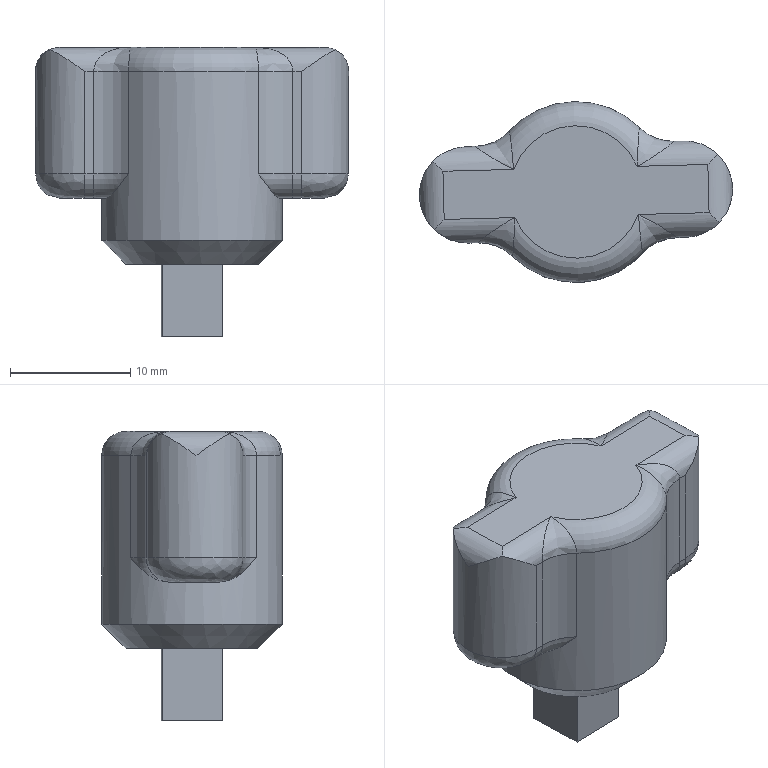Component | NX | WRENCH | 1 solid | 43 faces | volume 4195 mm3 | cylinder 17 | plane 13 | torus 6 | spline 6 | cone 1 | commonest cylinder face diameters 4 x10 8 x6 15 x1